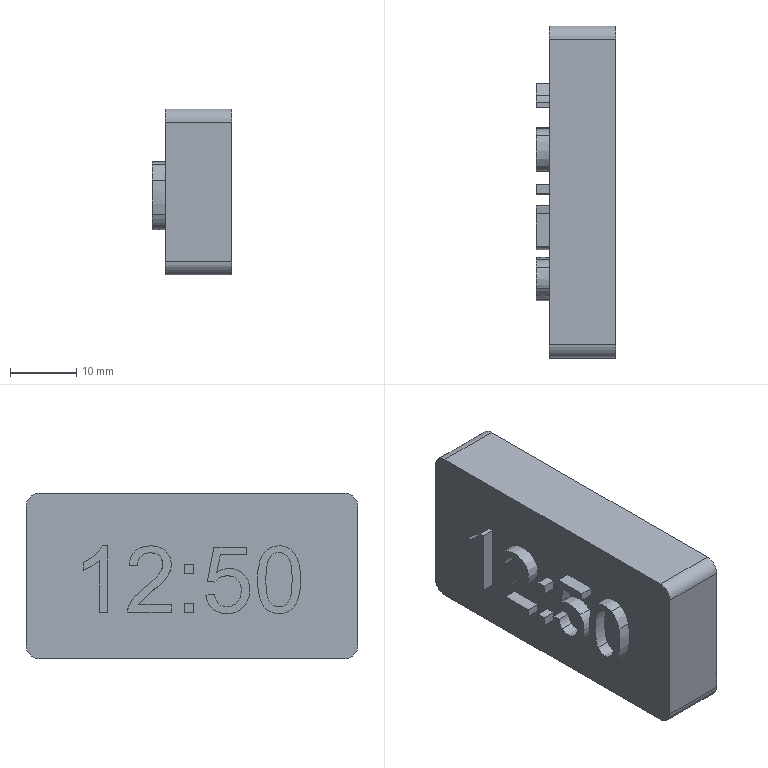Component | NX | DIGITALCLOCK1 | 1 solid | 72 faces | volume 12668 mm3 | plane 37 | other 31 | cylinder 4 | commonest cylinder face diameters 4 x4